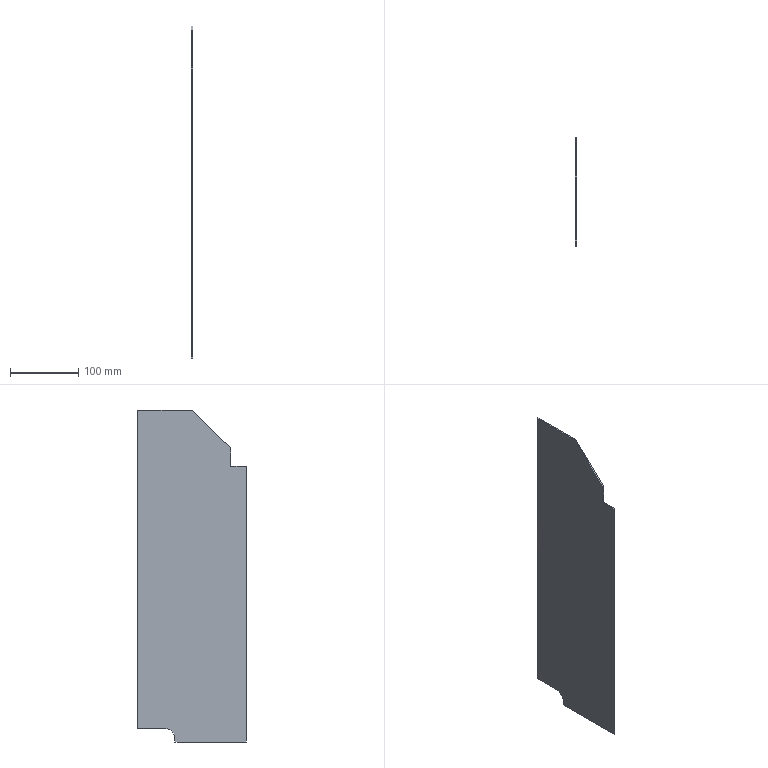Component | SolidWorks | LowerBaffle-2 | 1 solid | 12 faces | box 2 x 160 x 488 mm | volume 147032 mm3 | plane 11 | cylinder 1 | commonest cylinder face diameters 30 x1
build123d program:
from build123d import *

# Parameters (mm, degrees)
SKETCH1_W           = 488
SKETCH1_H           = 160
BOSS_EXTRUDE1_DEPTH = 2
CUT_EXTRUDE1_DEPTH  = 2
SKETCH3_W           = 20
SKETCH3_H           = 55
CUT_EXTRUDE2_DEPTH  = 2
FILLET1_R           = 15


with BuildPart() as part:
    # Sketch1 → Boss-Extrude1 (new body)
    with BuildSketch(Plane.XY):
        with Locations((115.965, -67.236)):
            Rectangle(SKETCH1_W, SKETCH1_H)
    extrude(amount=BOSS_EXTRUDE1_DEPTH)

    # Sketch2 → Cut-Extrude1 (cut)
    with BuildSketch(Plane.XY.offset(2)):
        Polygon((-128.035, -66.58), (-72.412, -124.236), (-45.035, -124.236), (-45.035, -147.236), (-128.035, -147.236), align=None)
    extrude(amount=-CUT_EXTRUDE1_DEPTH, mode=Mode.SUBTRACT)

    # Sketch3 → Cut-Extrude2 (cut)
    with BuildSketch(Plane.XY.offset(2)):
        with Locations((349.965, -14.736)):
            Rectangle(SKETCH3_W, SKETCH3_H)
    extrude(amount=-CUT_EXTRUDE2_DEPTH, mode=Mode.SUBTRACT)

    # Fillet1
    fillet1_edges = [part.edges().sort_by_distance(p)[0] for p in [
        (339.965, -42.236, 1),
    ]]
    fillet(fillet1_edges, radius=FILLET1_R)


solid = part.part

# Placed as in the assembly
solid = solid.moved(Location((-299.55, -391.198, 348.444), (0, 90, 0)))
STEP:
#1=COLOUR_RGB('',0.7922,0.8196,0.9333);
#2=FILL_AREA_STYLE_COLOUR('',#1);
#3=FILL_AREA_STYLE('',(#2));
#4=SURFACE_STYLE_FILL_AREA(#3);
#5=SURFACE_SIDE_STYLE('',(#4));
#6=SURFACE_STYLE_USAGE(.BOTH.,#5);
#7=PRESENTATION_STYLE_ASSIGNMENT((#6));
#8=CARTESIAN_POINT('',(-11.793,-14.899,18.759));
#9=VERTEX_POINT('',#8);
#10=CARTESIAN_POINT('',(-11.793,-18.023,18.759));
#11=VERTEX_POINT('',#10);
#12=CARTESIAN_POINT('',(-11.793,-14.899,18.759));
#13=DIRECTION('',(0.,-1.,-0.));
#14=VECTOR('',#13,39.37);
#15=LINE('',#12,#14);
#16=EDGE_CURVE('',#9,#11,#15,.T.);
#17=ORIENTED_EDGE('',*,*,#16,.T.);
#18=CARTESIAN_POINT('',(-11.715,-18.023,18.759));
#19=VERTEX_POINT('',#18);
#20=CARTESIAN_POINT('',(-11.793,-18.023,18.759));
#21=DIRECTION('',(1.,-0.,0.));
#22=VECTOR('',#21,39.37);
#23=LINE('',#20,#22);
#24=EDGE_CURVE('',#11,#19,#23,.T.);
#25=ORIENTED_EDGE('',*,*,#24,.T.);
#26=CARTESIAN_POINT('',(-11.715,-14.899,18.759));
#27=VERTEX_POINT('',#26);
#28=CARTESIAN_POINT('',(-11.715,-14.899,18.759));
#29=DIRECTION('',(0.,-1.,-0.));
#30=VECTOR('',#29,39.37);
#31=LINE('',#28,#30);
#32=EDGE_CURVE('',#27,#19,#31,.T.);
#33=ORIENTED_EDGE('',*,*,#32,.F.);
#34=CARTESIAN_POINT('',(-11.715,-14.899,18.759));
#35=DIRECTION('',(-1.,0.,-0.));
#36=VECTOR('',#35,39.37);
#37=LINE('',#34,#36);
#38=EDGE_CURVE('',#27,#9,#37,.T.);
#39=ORIENTED_EDGE('',*,*,#38,.T.);
#40=EDGE_LOOP('',(#17,#25,#33,#39));
#41=FACE_OUTER_BOUND('',#40,.T.);
#42=CARTESIAN_POINT('',(-11.715,-14.899,18.759));
#43=DIRECTION('',(0.,0.,-1.));
#44=DIRECTION('',(-0.,1.,0.));
#45=AXIS2_PLACEMENT_3D('',#42,#43,#44);
#46=PLANE('',#45);
#47=ADVANCED_FACE('',(#41),#46,.F.);
#48=CARTESIAN_POINT('',(-11.715,-21.198,15.491));
#49=VERTEX_POINT('',#48);
#50=CARTESIAN_POINT('',(-11.715,-21.198,-0.4536));
#51=VERTEX_POINT('',#50);
#52=CARTESIAN_POINT('',(-11.715,-21.198,18.759));
#53=DIRECTION('',(0.,-0.,-1.));
#54=VECTOR('',#53,39.37);
#55=LINE('',#52,#54);
#56=EDGE_CURVE('',#49,#51,#55,.T.);
#57=ORIENTED_EDGE('',*,*,#56,.F.);
#58=CARTESIAN_POINT('',(-11.793,-21.198,15.491));
#59=VERTEX_POINT('',#58);
#60=CARTESIAN_POINT('',(-11.793,-21.198,15.491));
#61=DIRECTION('',(1.,-0.,0.));
#62=VECTOR('',#61,39.37);
#63=LINE('',#60,#62);
#64=EDGE_CURVE('',#59,#49,#63,.T.);
#65=ORIENTED_EDGE('',*,*,#64,.F.);
#66=CARTESIAN_POINT('',(-11.793,-21.198,-0.4536));
#67=VERTEX_POINT('',#66);
#68=CARTESIAN_POINT('',(-11.793,-21.198,18.759));
#69=DIRECTION('',(0.,-0.,-1.));
#70=VECTOR('',#69,39.37);
#71=LINE('',#68,#70);
#72=EDGE_CURVE('',#59,#67,#71,.T.);
#73=ORIENTED_EDGE('',*,*,#72,.T.);
#74=CARTESIAN_POINT('',(-11.715,-21.198,-0.4536));
#75=DIRECTION('',(-1.,0.,-0.));
#76=VECTOR('',#75,39.37);
#77=LINE('',#74,#76);
#78=EDGE_CURVE('',#51,#67,#77,.T.);
#79=ORIENTED_EDGE('',*,*,#78,.F.);
#80=EDGE_LOOP('',(#57,#65,#73,#79));
#81=FACE_OUTER_BOUND('',#80,.T.);
#82=CARTESIAN_POINT('',(-11.715,-21.198,18.759));
#83=DIRECTION('',(0.,1.,-0.));
#84=DIRECTION('',(1.,-0.,0.));
#85=AXIS2_PLACEMENT_3D('',#82,#83,#84);
#86=PLANE('',#85);
#87=ADVANCED_FACE('',(#81),#86,.F.);
#88=CARTESIAN_POINT('',(-11.793,-17.064,-0.4536));
#89=VERTEX_POINT('',#88);
#90=CARTESIAN_POINT('',(-11.793,-14.899,-0.4536));
#91=DIRECTION('',(-0.,1.,0.));
#92=VECTOR('',#91,39.37);
#93=LINE('',#90,#92);
#94=EDGE_CURVE('',#67,#89,#93,.T.);
#95=ORIENTED_EDGE('',*,*,#94,.T.);
#96=CARTESIAN_POINT('',(-11.715,-17.064,-0.4536));
#97=VERTEX_POINT('',#96);
#98=CARTESIAN_POINT('',(-11.793,-17.064,-0.4536));
#99=DIRECTION('',(1.,-0.,0.));
#100=VECTOR('',#99,39.37);
#101=LINE('',#98,#100);
#102=EDGE_CURVE('',#89,#97,#101,.T.);
#103=ORIENTED_EDGE('',*,*,#102,.T.);
#104=CARTESIAN_POINT('',(-11.715,-14.899,-0.4536));
#105=DIRECTION('',(-0.,1.,0.));
#106=VECTOR('',#105,39.37);
#107=LINE('',#104,#106);
#108=EDGE_CURVE('',#51,#97,#107,.T.);
#109=ORIENTED_EDGE('',*,*,#108,.F.);
#110=ORIENTED_EDGE('',*,*,#78,.T.);
#111=EDGE_LOOP('',(#95,#103,#109,#110));
#112=FACE_OUTER_BOUND('',#111,.T.);
#113=CARTESIAN_POINT('',(-11.715,-14.899,-0.4536));
#114=DIRECTION('',(-0.,-0.,1.));
#115=DIRECTION('',(0.,-1.,-0.));
#116=AXIS2_PLACEMENT_3D('',#113,#114,#115);
#117=PLANE('',#116);
#118=ADVANCED_FACE('',(#112),#117,.F.);
#119=CARTESIAN_POINT('',(-11.715,-14.899,0.3338));
#120=VERTEX_POINT('',#119);
#121=CARTESIAN_POINT('',(-11.715,-14.899,18.759));
#122=DIRECTION('',(-0.,0.,1.));
#123=VECTOR('',#122,39.37);
#124=LINE('',#121,#123);
#125=EDGE_CURVE('',#120,#27,#124,.T.);
#126=ORIENTED_EDGE('',*,*,#125,.F.);
#127=CARTESIAN_POINT('',(-11.793,-14.899,0.3338));
#128=VERTEX_POINT('',#127);
#129=CARTESIAN_POINT('',(-11.793,-14.899,0.3338));
#130=DIRECTION('',(1.,-0.,0.));
#131=VECTOR('',#130,39.37);
#132=LINE('',#129,#131);
#133=EDGE_CURVE('',#128,#120,#132,.T.);
#134=ORIENTED_EDGE('',*,*,#133,.F.);
#135=CARTESIAN_POINT('',(-11.793,-14.899,18.759));
#136=DIRECTION('',(-0.,0.,1.));
#137=VECTOR('',#136,39.37);
#138=LINE('',#135,#137);
#139=EDGE_CURVE('',#128,#9,#138,.T.);
#140=ORIENTED_EDGE('',*,*,#139,.T.);
#141=ORIENTED_EDGE('',*,*,#38,.F.);
#142=EDGE_LOOP('',(#126,#134,#140,#141));
#143=FACE_OUTER_BOUND('',#142,.T.);
#144=CARTESIAN_POINT('',(-11.715,-14.899,18.759));
#145=DIRECTION('',(-0.,-1.,0.));
#146=DIRECTION('',(-1.,0.,-0.));
#147=AXIS2_PLACEMENT_3D('',#144,#145,#146);
#148=PLANE('',#147);
#149=ADVANCED_FACE('',(#143),#148,.F.);
#150=CARTESIAN_POINT('',(-11.715,-17.064,-0.2567));
#151=VERTEX_POINT('',#150);
#152=CARTESIAN_POINT('',(-11.715,-17.064,-0.4536));
#153=DIRECTION('',(0.,-0.,-1.));
#154=VECTOR('',#153,39.37);
#155=LINE('',#152,#154);
#156=EDGE_CURVE('',#151,#97,#155,.T.);
#157=ORIENTED_EDGE('',*,*,#156,.F.);
#158=CARTESIAN_POINT('',(-11.715,-16.474,0.3338));
#159=VERTEX_POINT('',#158);
#160=CARTESIAN_POINT('',(-11.715,-16.474,-0.2567));
#161=DIRECTION('',(-1.,0.,-0.));
#162=DIRECTION('',(0.,0.,-1.));
#163=AXIS2_PLACEMENT_3D('',#160,#161,#162);
#164=CIRCLE('',#163,0.5906);
#165=EDGE_CURVE('',#151,#159,#164,.T.);
#166=ORIENTED_EDGE('',*,*,#165,.T.);
#167=CARTESIAN_POINT('',(-11.715,-14.899,0.3338));
#168=DIRECTION('',(0.,-1.,0.));
#169=VECTOR('',#168,39.37);
#170=LINE('',#167,#169);
#171=EDGE_CURVE('',#120,#159,#170,.T.);
#172=ORIENTED_EDGE('',*,*,#171,.F.);
#173=ORIENTED_EDGE('',*,*,#125,.T.);
#174=ORIENTED_EDGE('',*,*,#32,.T.);
#175=CARTESIAN_POINT('',(-11.715,-20.293,16.569));
#176=VERTEX_POINT('',#175);
#177=CARTESIAN_POINT('',(-11.715,-18.023,18.759));
#178=DIRECTION('',(-0.,0.7197,0.6943));
#179=VECTOR('',#178,39.37);
#180=LINE('',#177,#179);
#181=EDGE_CURVE('',#176,#19,#180,.T.);
#182=ORIENTED_EDGE('',*,*,#181,.F.);
#183=CARTESIAN_POINT('',(-11.715,-20.293,15.491));
#184=VERTEX_POINT('',#183);
#185=CARTESIAN_POINT('',(-11.715,-20.293,16.569));
#186=DIRECTION('',(-0.,0.,1.));
#187=VECTOR('',#186,39.37);
#188=LINE('',#185,#187);
#189=EDGE_CURVE('',#184,#176,#188,.T.);
#190=ORIENTED_EDGE('',*,*,#189,.F.);
#191=CARTESIAN_POINT('',(-11.715,-20.293,15.491));
#192=DIRECTION('',(-0.,1.,0.));
#193=VECTOR('',#192,39.37);
#194=LINE('',#191,#193);
#195=EDGE_CURVE('',#49,#184,#194,.T.);
#196=ORIENTED_EDGE('',*,*,#195,.F.);
#197=ORIENTED_EDGE('',*,*,#56,.T.);
#198=ORIENTED_EDGE('',*,*,#108,.T.);
#199=EDGE_LOOP('',(#157,#166,#172,#173,#174,#182,#190,#196,#197,#198));
#200=FACE_OUTER_BOUND('',#199,.T.);
#201=CARTESIAN_POINT('',(-11.715,-15.401,13.718));
#202=DIRECTION('',(1.,-0.,0.));
#203=DIRECTION('',(0.,-0.,-1.));
#204=AXIS2_PLACEMENT_3D('',#201,#202,#203);
#205=PLANE('',#204);
#206=ADVANCED_FACE('',(#200),#205,.T.);
#207=CARTESIAN_POINT('',(-11.793,-16.474,0.3338));
#208=VERTEX_POINT('',#207);
#209=CARTESIAN_POINT('',(-11.793,-14.899,0.3338));
#210=DIRECTION('',(0.,-1.,0.));
#211=VECTOR('',#210,39.37);
#212=LINE('',#209,#211);
#213=EDGE_CURVE('',#128,#208,#212,.T.);
#214=ORIENTED_EDGE('',*,*,#213,.T.);
#215=CARTESIAN_POINT('',(-11.793,-17.064,-0.2567));
#216=VERTEX_POINT('',#215);
#217=CARTESIAN_POINT('',(-11.793,-16.474,-0.2567));
#218=DIRECTION('',(1.,-0.,0.));
#219=DIRECTION('',(0.,0.,-1.));
#220=AXIS2_PLACEMENT_3D('',#217,#218,#219);
#221=CIRCLE('',#220,0.5906);
#222=EDGE_CURVE('',#208,#216,#221,.T.);
#223=ORIENTED_EDGE('',*,*,#222,.T.);
#224=CARTESIAN_POINT('',(-11.793,-17.064,-0.4536));
#225=DIRECTION('',(0.,-0.,-1.));
#226=VECTOR('',#225,39.37);
#227=LINE('',#224,#226);
#228=EDGE_CURVE('',#216,#89,#227,.T.);
#229=ORIENTED_EDGE('',*,*,#228,.T.);
#230=ORIENTED_EDGE('',*,*,#94,.F.);
#231=ORIENTED_EDGE('',*,*,#72,.F.);
#232=CARTESIAN_POINT('',(-11.793,-20.293,15.491));
#233=VERTEX_POINT('',#232);
#234=CARTESIAN_POINT('',(-11.793,-20.293,15.491));
#235=DIRECTION('',(-0.,1.,0.));
#236=VECTOR('',#235,39.37);
#237=LINE('',#234,#236);
#238=EDGE_CURVE('',#59,#233,#237,.T.);
#239=ORIENTED_EDGE('',*,*,#238,.T.);
#240=CARTESIAN_POINT('',(-11.793,-20.293,16.569));
#241=VERTEX_POINT('',#240);
#242=CARTESIAN_POINT('',(-11.793,-20.293,16.569));
#243=DIRECTION('',(-0.,0.,1.));
#244=VECTOR('',#243,39.37);
#245=LINE('',#242,#244);
#246=EDGE_CURVE('',#233,#241,#245,.T.);
#247=ORIENTED_EDGE('',*,*,#246,.T.);
#248=CARTESIAN_POINT('',(-11.793,-18.023,18.759));
#249=DIRECTION('',(-0.,0.7197,0.6943));
#250=VECTOR('',#249,39.37);
#251=LINE('',#248,#250);
#252=EDGE_CURVE('',#241,#11,#251,.T.);
#253=ORIENTED_EDGE('',*,*,#252,.T.);
#254=ORIENTED_EDGE('',*,*,#16,.F.);
#255=ORIENTED_EDGE('',*,*,#139,.F.);
#256=EDGE_LOOP('',(#214,#223,#229,#230,#231,#239,#247,#253,#254,#255));
#257=FACE_OUTER_BOUND('',#256,.T.);
#258=CARTESIAN_POINT('',(-11.793,-15.401,13.718));
#259=DIRECTION('',(1.,-0.,0.));
#260=DIRECTION('',(0.,-0.,-1.));
#261=AXIS2_PLACEMENT_3D('',#258,#259,#260);
#262=PLANE('',#261);
#263=ADVANCED_FACE('',(#257),#262,.F.);
#264=ORIENTED_EDGE('',*,*,#181,.T.);
#265=ORIENTED_EDGE('',*,*,#24,.F.);
#266=ORIENTED_EDGE('',*,*,#252,.F.);
#267=CARTESIAN_POINT('',(-11.793,-20.293,16.569));
#268=DIRECTION('',(1.,-0.,0.));
#269=VECTOR('',#268,39.37);
#270=LINE('',#267,#269);
#271=EDGE_CURVE('',#241,#176,#270,.T.);
#272=ORIENTED_EDGE('',*,*,#271,.T.);
#273=EDGE_LOOP('',(#264,#265,#266,#272));
#274=FACE_OUTER_BOUND('',#273,.T.);
#275=CARTESIAN_POINT('',(-11.793,-18.023,18.759));
#276=DIRECTION('',(-0.,0.6943,-0.7197));
#277=DIRECTION('',(-0.,0.7197,0.6943));
#278=AXIS2_PLACEMENT_3D('',#275,#276,#277);
#279=PLANE('',#278);
#280=ADVANCED_FACE('',(#274),#279,.F.);
#281=ORIENTED_EDGE('',*,*,#189,.T.);
#282=ORIENTED_EDGE('',*,*,#271,.F.);
#283=ORIENTED_EDGE('',*,*,#246,.F.);
#284=CARTESIAN_POINT('',(-11.793,-20.293,15.491));
#285=DIRECTION('',(1.,-0.,0.));
#286=VECTOR('',#285,39.37);
#287=LINE('',#284,#286);
#288=EDGE_CURVE('',#233,#184,#287,.T.);
#289=ORIENTED_EDGE('',*,*,#288,.T.);
#290=EDGE_LOOP('',(#281,#282,#283,#289));
#291=FACE_OUTER_BOUND('',#290,.T.);
#292=CARTESIAN_POINT('',(-11.793,-20.293,16.569));
#293=DIRECTION('',(0.,1.,-0.));
#294=DIRECTION('',(1.,-0.,0.));
#295=AXIS2_PLACEMENT_3D('',#292,#293,#294);
#296=PLANE('',#295);
#297=ADVANCED_FACE('',(#291),#296,.F.);
#298=ORIENTED_EDGE('',*,*,#195,.T.);
#299=ORIENTED_EDGE('',*,*,#288,.F.);
#300=ORIENTED_EDGE('',*,*,#238,.F.);
#301=ORIENTED_EDGE('',*,*,#64,.T.);
#302=EDGE_LOOP('',(#298,#299,#300,#301));
#303=FACE_OUTER_BOUND('',#302,.T.);
#304=CARTESIAN_POINT('',(-11.793,-20.293,15.491));
#305=DIRECTION('',(0.,0.,-1.));
#306=DIRECTION('',(-0.,1.,0.));
#307=AXIS2_PLACEMENT_3D('',#304,#305,#306);
#308=PLANE('',#307);
#309=ADVANCED_FACE('',(#303),#308,.F.);
#310=ORIENTED_EDGE('',*,*,#228,.F.);
#311=CARTESIAN_POINT('',(-11.715,-17.064,-0.2567));
#312=DIRECTION('',(1.,-0.,0.));
#313=VECTOR('',#312,39.37);
#314=LINE('',#311,#313);
#315=EDGE_CURVE('',#216,#151,#314,.T.);
#316=ORIENTED_EDGE('',*,*,#315,.T.);
#317=ORIENTED_EDGE('',*,*,#156,.T.);
#318=ORIENTED_EDGE('',*,*,#102,.F.);
#319=EDGE_LOOP('',(#310,#316,#317,#318));
#320=FACE_OUTER_BOUND('',#319,.T.);
#321=CARTESIAN_POINT('',(-11.793,-17.064,-0.4536));
#322=DIRECTION('',(-0.,-1.,0.));
#323=DIRECTION('',(-1.,0.,-0.));
#324=AXIS2_PLACEMENT_3D('',#321,#322,#323);
#325=PLANE('',#324);
#326=ADVANCED_FACE('',(#320),#325,.F.);
#327=ORIENTED_EDGE('',*,*,#171,.T.);
#328=CARTESIAN_POINT('',(-11.793,-16.474,0.3338));
#329=DIRECTION('',(-1.,0.,-0.));
#330=VECTOR('',#329,39.37);
#331=LINE('',#328,#330);
#332=EDGE_CURVE('',#159,#208,#331,.T.);
#333=ORIENTED_EDGE('',*,*,#332,.T.);
#334=ORIENTED_EDGE('',*,*,#213,.F.);
#335=ORIENTED_EDGE('',*,*,#133,.T.);
#336=EDGE_LOOP('',(#327,#333,#334,#335));
#337=FACE_OUTER_BOUND('',#336,.T.);
#338=CARTESIAN_POINT('',(-11.793,-14.899,0.3338));
#339=DIRECTION('',(-0.,0.,1.));
#340=DIRECTION('',(1.,-0.,0.));
#341=AXIS2_PLACEMENT_3D('',#338,#339,#340);
#342=PLANE('',#341);
#343=ADVANCED_FACE('',(#337),#342,.F.);
#344=ORIENTED_EDGE('',*,*,#222,.F.);
#345=ORIENTED_EDGE('',*,*,#332,.F.);
#346=ORIENTED_EDGE('',*,*,#165,.F.);
#347=ORIENTED_EDGE('',*,*,#315,.F.);
#348=EDGE_LOOP('',(#344,#345,#346,#347));
#349=FACE_OUTER_BOUND('',#348,.T.);
#350=CARTESIAN_POINT('',(-11.793,-16.474,-0.2567));
#351=DIRECTION('',(-1.,0.,-0.));
#352=DIRECTION('',(0.,0.,1.));
#353=AXIS2_PLACEMENT_3D('',#350,#351,#352);
#354=CYLINDRICAL_SURFACE('',#353,0.5906);
#355=ADVANCED_FACE('',(#349),#354,.F.);
#356=CLOSED_SHELL('',(#47,#87,#118,#149,#206,#263,#280,#297,#309,#326,#343,#355));
#357=MANIFOLD_SOLID_BREP('',#356);
#358=STYLED_ITEM('',(#7),#357);
#359=PRESENTATION_LAYER_ASSIGNMENT('','',(#358));
#360=CARTESIAN_POINT('',(0.,0.,0.));
#361=DIRECTION('',(0.,0.,1.));
#362=DIRECTION('',(1.,0.,0.));
#363=AXIS2_PLACEMENT_3D('',#360,#361,#362);
#364=(LENGTH_UNIT()NAMED_UNIT(*)SI_UNIT($,.METRE.));
#365=LENGTH_MEASURE_WITH_UNIT(LENGTH_MEASURE(0.0254),#364);
#366=DIMENSIONAL_EXPONENTS(1.,0.,0.,0.,0.,0.,0.);
#367=(CONVERSION_BASED_UNIT('',#365)LENGTH_UNIT()NAMED_UNIT(#366));
#368=UNCERTAINTY_MEASURE_WITH_UNIT(LENGTH_MEASURE(0.00001),#367,'','');
#369=(NAMED_UNIT(*)PLANE_ANGLE_UNIT()SI_UNIT($,.RADIAN.));
#370=(NAMED_UNIT(*)SI_UNIT($,.STERADIAN.)SOLID_ANGLE_UNIT());
#371=(GEOMETRIC_REPRESENTATION_CONTEXT(3)GLOBAL_UNCERTAINTY_ASSIGNED_CONTEXT((#368))GLOBAL_UNIT_ASSIGNED_CONTEXT((#367,#369,#370))REPRESENTATION_CONTEXT('',''));
#372=ADVANCED_BREP_SHAPE_REPRESENTATION('',(#357,#363),#371);
#373=(LENGTH_UNIT()NAMED_UNIT(*)SI_UNIT($,.METRE.));
#374=LENGTH_MEASURE_WITH_UNIT(LENGTH_MEASURE(0.0254),#373);
#375=DIMENSIONAL_EXPONENTS(1.,0.,0.,0.,0.,0.,0.);
#376=(CONVERSION_BASED_UNIT('',#374)LENGTH_UNIT()NAMED_UNIT(#375));
#377=UNCERTAINTY_MEASURE_WITH_UNIT(LENGTH_MEASURE(0.00001),#376,'','');
#378=(NAMED_UNIT(*)PLANE_ANGLE_UNIT()SI_UNIT($,.RADIAN.));
#379=(NAMED_UNIT(*)SI_UNIT($,.STERADIAN.)SOLID_ANGLE_UNIT());
#380=(GEOMETRIC_REPRESENTATION_CONTEXT(3)GLOBAL_UNCERTAINTY_ASSIGNED_CONTEXT((#377))GLOBAL_UNIT_ASSIGNED_CONTEXT((#376,#378,#379))REPRESENTATION_CONTEXT('',''));
#381=MECHANICAL_DESIGN_GEOMETRIC_PRESENTATION_REPRESENTATION('',(#358),#380);